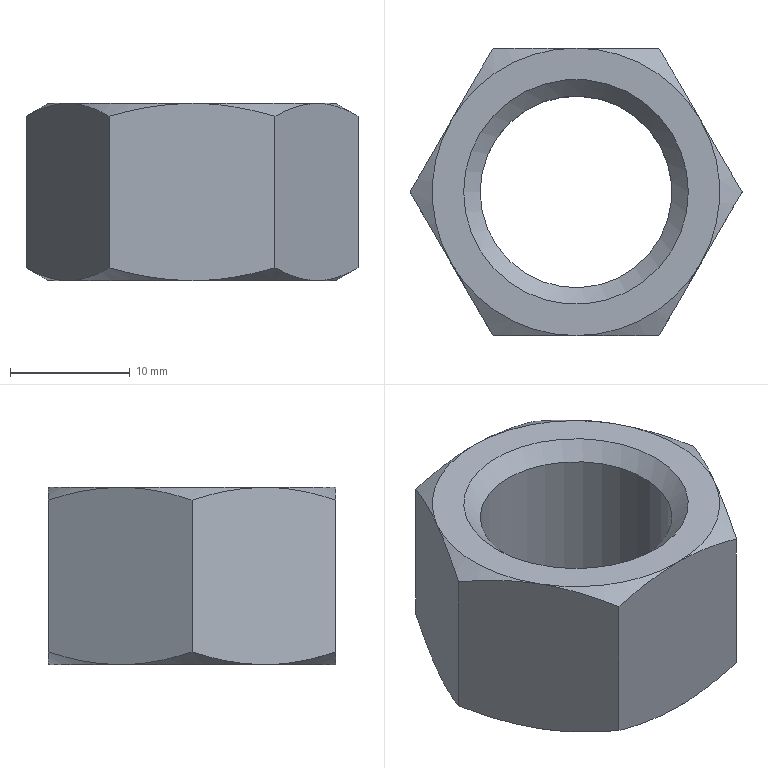Component | NX | GB-T6170_F-2000_M16X2 | 1 solid | 23 faces | volume 4275 mm3 | cone 14 | plane 8 | cylinder 1 | commonest cylinder face diameters 16 x1